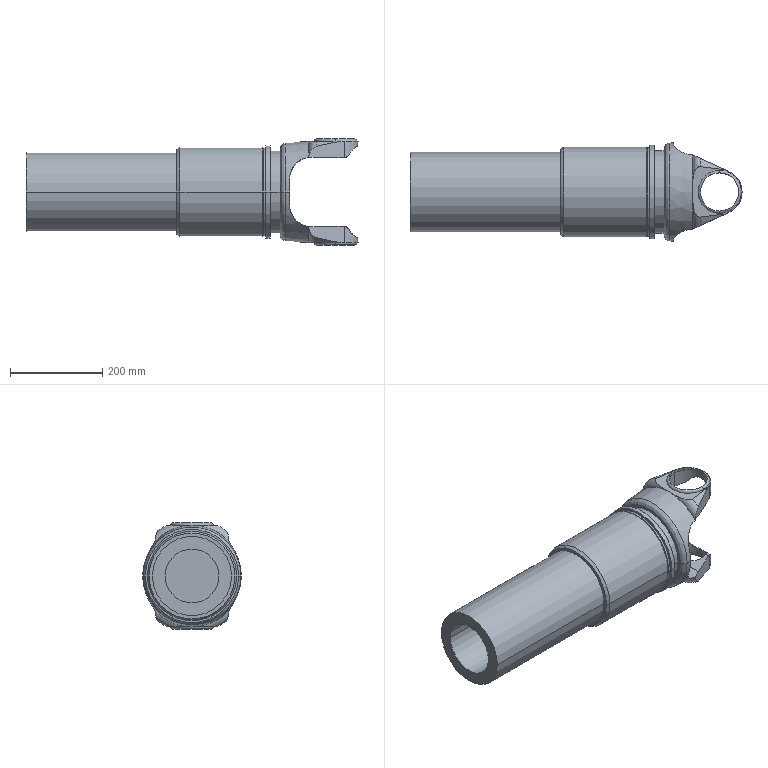Component | NX | BRAZO_HUECO_PREDETERMINADO_COMO_MECANIZADA | 3 solids | 69 faces | volume 11604253 mm3 | cylinder 32 | plane 19 | torus 10 | cone 8 | commonest cylinder face diameters 83 x8 30 x4 116.772 x2 171.397 x2 193.579 x2 187.019 x2 191.308 x2 201.927 x2